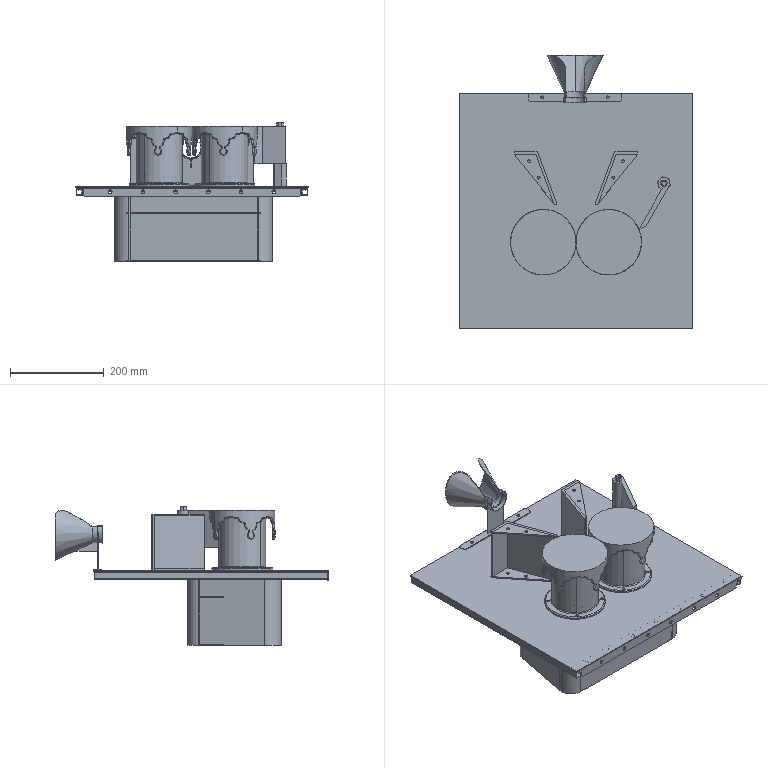Assembly | SolidWorks | mm | 23 component files | 28 solids | 1527 faces | box 500 x 585 x 297 mm | volume 2981683 mm3 | cylinder 716 | plane 629 | spline 90 | sphere 64 | torus 24 | cone 4 | commonest cylinder face diameters 2 x304 130 x118 6 x36 10 x28 15 x28 8 x26 4 x24 60 x24
Bill of materials:
AngleIron2 | 1 |  | Long, straight, equal-leg L-shaped angle profile. Both legs have evenly spaced round holes, and the ends have angled cuts with small semicircular notches.
Baffle | 2 |  | Thick, extruded triangular prism with small rounded corners and two round holes through the triangular face.
Column | 2 |  | Long, straight, hollow tube with a square cross-section and uniform wall thickness.
DoughGuideFunnel | 1 |  | Flared, horn-like conical body with a U-shaped slot cut into it. It has a stepped cylindrical collar at the narrow end and sits on a flat web that stands on a thin strip with rounded ends and two holes.
DriveGuard | 1 |  | Open rectangular box or tray with rounded vertical corners and a thin flange around the top rim. The flange has four corner holes, and there is a small hole in the floor.
ExcessDoughCuttingWheelBearing | 4 |  | Flat annular disc (washer-like ring) with a central through hole. One face has a concentric annular groove that leaves a raised ring around the bore.
FormingWheel | 2 |  | Round, flat-topped disc with an irregular, drip-shaped thin skirt hanging from its edge, and a slender cylindrical rod extending down from the centre.
FormingWheelMotor | 1 |  | Square prismatic block with concave rounded cut-outs along all four vertical corner edges. A cylindrical shaft with a raised key-like feature sticks out from a shallow circular boss on the top face.
FormingWheelMountingCover | 2 |  | Cylindrical cup- or housing-like body on a wider circular base flange with four round holes. The top face has a circular recess with a smaller central hole.
FrameSidePlate2 | 1 |  | Thin, flat square sheet or plate with three small round through holes: two of similar size and one smaller.
M10Screw | 1 |  | Cylindrical pin with a larger cylindrical head containing a hexagonal socket, and a long, plain, smooth shank. Resembles a socket-head cap screw.
Scraper | 1 |  | Flat rectangular leaf with a cylindrical knuckle along one edge containing a round through bore, and an angled cut at the opposite end. Resembles a hinge leaf.
ScraperSupport | 1 |  | Elongated hexagonal prism with a single centered circular through-bore along its long axis; shaped like a hex spacer or standoff.
SmallPulley1 | 2 |  | Thin, flat spur-gear-like disc with many straight-cut external teeth, about 50 (approximate count), and a small central bore with two small notches on opposite sides.
SmallPulley3 | 1 |  | Thick spur-gear-like part with about 16 coarse, pointed straight-cut teeth and a central circular bore with one rectangular keyway slot.
Mates:
1. coincident | Baffle-1 face at (184.241, -164.715, 1590.724) dir (0, 1, 0) | Baffle-2 face at (448.241, -164.715, 1470.724) dir (0, 1, 0)
2. gear | SmallPulley1-4 sketch segment at (386.241, -358.715, 1455.724) dir (0, 0, 1) r 70 | SmallPulley1-5 sketch segment at (246.241, -358.715, 1455.724) dir (0, 0, 1) r 70
3. coincident | SmallPulley1-5 face at (246.241, -358.715, 1435.724) dir (0, 0, -1) | SmallPulley3-1 face at (246.241, -267.715, 1435.724) dir (0, 0, -1)
4. gear | SmallPulley3-1 sketch segment at (246.241, -267.715, 1455.724) dir (0, 0, 1) r 18 | SmallPulley1-5 sketch segment at (246.241, -358.715, 1455.724) dir (0, 0, 1) r 70
5. concentric | SmallPulley3-1 face at (246.241, -267.715, 1410.724) dir (0, 0, 1) r 5 | FormingWheelMotor-1 face at (246.241, -267.715, 1410.724) dir (0, 0, 1) r 5
6. coincident | SmallPulley3-1 face at (246.241, -267.715, 1455.724) dir (0, 0, 1) | FormingWheelMotor-1 face at (246.241, -267.715, 1455.724) dir (0, 0, 1)
7. coincident | FrameSidePlate2-1 face at (316.241, -291.715, 1470.724) dir (0, 0, 1) | Baffle-1 face at (234.241, -164.715, 1470.724) dir (0, 0, -1)
8. coincident | FrameSidePlate2-1 face at (316.241, -291.715, 1470.724) dir (0, 0, 1) | Baffle-2 face at (398.241, -164.715, 1470.724) dir (0, 0, -1)
9. coincident | FrameSidePlate2-1 edge at (66.241, -39.715, 1470.724) dir (1, 0, 0) | DoughGuideFunnel-1 face at (414.241, -39.715, 1470.724) dir (0, 1, 0)
10. parallel | FrameSidePlate2-1 face at (316.241, -291.715, 1470.724) dir (0, 0, 1) | DoughGuideFunnel-1 face at (314.241, 41.285, 1470.724) dir (0, 0, -1)
11. concentric | ScraperSupport-1 face at (504.241, -232.715, 1470.724) dir (0, 0, 1) r 5 | Scraper-1 face at (504.241, -232.715, 1518.724) dir (0, 0, 1) r 5
12. coincident | ScraperSupport-1 face at (504.241, -232.715, 1518.724) dir (0, 0, 1) | Scraper-1 face at (504.241, -232.715, 1518.724) dir (0, 0, -1)
13. concentric | Scraper-1 face at (504.241, -232.715, 1518.724) dir (0, 0, 1) r 5 | M10Screw-1 face at (504.241, -232.715, 1598.724) dir (0, 0, -1) r 5
14. coincident | Scraper-1 face at (504.241, -232.715, 1598.724) dir (0, 0, 1) | M10Screw-1 face at (504.241, -232.715, 1598.724) dir (0, 0, -1)
15. coincident | FrameSidePlate2-1 face at (316.241, -291.715, 1470.724) dir (0, 0, 1) | ScraperSupport-1 face at (504.241, -232.715, 1470.724) dir (0, 0, -1)
16. coincident | FormingWheelMountingCover-3 face at (386.241, -358.715, 1590.724) dir (0, 0, 1) | ExcessDoughCuttingWheelBearing-5 face at (397.598, -345.401, 1590.724) dir (0, 0, 1)
17. concentric | FormingWheelMountingCover-3 face at (386.241, -358.715, 1582.724) dir (0, 0, 1) r 22.5 | ExcessDoughCuttingWheelBearing-5 face at (386.241, -358.715, 1592.181) dir (0, 0, 1) r 22.5
18. distance | FormingWheelMountingCover-3 face at (386.241, -358.715, 1590.724) dir (0, 0, 1) | FormingWheel-3 face at (386.241, -358.715, 1595.724) dir (0, 0, -1)
19. coincident | FormingWheelMountingCover-3 face at (386.241, -358.715, 1490.724) dir (0, 0, -1) | ExcessDoughCuttingWheelBearing-6 face at (397.598, -345.401, 1490.724) dir (0, 0, 1)
20. concentric | ExcessDoughCuttingWheelBearing-5 face at (386.241, -358.715, 1592.181) dir (0, 0, 1) r 7.5 | FormingWheel-3 face at (386.241, -358.715, 1435.724) dir (0, 0, 1) r 7.5
21. concentric | FormingWheel-3 face at (386.241, -358.715, 1435.724) dir (0, 0, 1) r 7.5 | ExcessDoughCuttingWheelBearing-6 face at (386.241, -358.715, 1492.181) dir (0, 0, 1) r 7.5
22. coincident | FormingWheelMountingCover-3 plane at (386.241, -358.715, 1580.724) dir (0.7608, -0.6489, 0) | SmallPulley1-4 plane at (386.241, -358.715, 1435.724) dir (0.7608, -0.6489, 0)
23. coincident | FrameSidePlate2-1 face at (316.241, -291.715, 1470.724) dir (0, 0, 1) | FormingWheelMountingCover-3 face at (386.241, -358.715, 1470.724) dir (0, 0, -1)
24. concentric | FormingWheel-3 face at (386.241, -358.715, 1435.724) dir (0, 0, 1) r 7.5 | SmallPulley1-4 face at (386.241, -358.715, 1410.724) dir (0, 0, 1) r 7.5
25. coincident | FormingWheel-3 face at (386.241, -358.715, 1435.724) dir (0, 0, -1) | SmallPulley1-4 face at (386.241, -358.715, 1435.724) dir (0, 0, -1)
26. coincident | FormingWheel-3 face at (386.241, -358.715, 1535.724) dir (0, 0, 1) r 70 | Scraper-1 edge at (450.713, -331.451, 1518.724) dir (0, 0, 1)
27. coincident | FormingWheelMountingCover-2 face at (246.241, -358.715, 1590.724) dir (0, 0, 1) | ExcessDoughCuttingWheelBearing-3 face at (257.598, -345.401, 1590.724) dir (0, 0, 1)
28. concentric | FormingWheelMountingCover-2 face at (246.241, -358.715, 1582.724) dir (0, 0, 1) r 22.5 | ExcessDoughCuttingWheelBearing-3 face at (246.241, -358.715, 1592.181) dir (0, 0, 1) r 22.5
29. distance | FormingWheelMountingCover-2 face at (246.241, -358.715, 1590.724) dir (0, 0, 1) | FormingWheel-2 face at (246.241, -358.715, 1595.724) dir (0, 0, -1)
30. coincident | FormingWheelMountingCover-2 face at (246.241, -358.715, 1490.724) dir (0, 0, -1) | ExcessDoughCuttingWheelBearing-4 face at (257.598, -345.401, 1490.724) dir (0, 0, 1)
31. concentric | ExcessDoughCuttingWheelBearing-3 face at (246.241, -358.715, 1592.181) dir (0, 0, 1) r 7.5 | FormingWheel-2 face at (246.241, -358.715, 1435.724) dir (0, 0, 1) r 7.5
32. concentric | FormingWheel-2 face at (246.241, -358.715, 1435.724) dir (0, 0, 1) r 7.5 | ExcessDoughCuttingWheelBearing-4 face at (246.241, -358.715, 1492.181) dir (0, 0, 1) r 7.5
33. coincident | FrameSidePlate2-1 face at (316.241, -291.715, 1470.724) dir (0, 0, 1) | FormingWheelMountingCover-2 face at (246.241, -358.715, 1470.724) dir (0, 0, -1)
34. concentric | FormingWheel-2 face at (246.241, -358.715, 1435.724) dir (0, 0, 1) r 7.5 | SmallPulley1-5 face at (246.241, -358.715, 1410.724) dir (0, 0, 1) r 7.5
35. coincident | FormingWheel-2 face at (246.241, -358.715, 1435.724) dir (0, 0, -1) | SmallPulley1-5 face at (246.241, -358.715, 1435.724) dir (0, 0, -1)
36. parallel | FormingWheel-2 plane at (271.112, -396.218, 1595.724) dir (0.5527, -0.8334, 0) | FormingWheel-3 plane at (411.112, -396.218, 1595.724) dir (0.5527, -0.8334, 0)
37. parallel | FormingWheel-2 plane at (271.112, -396.218, 1595.724) dir (0.5527, -0.8334, 0) | FormingWheel-3 plane at (411.112, -396.218, 1595.724) dir (0.5527, -0.8334, 0)